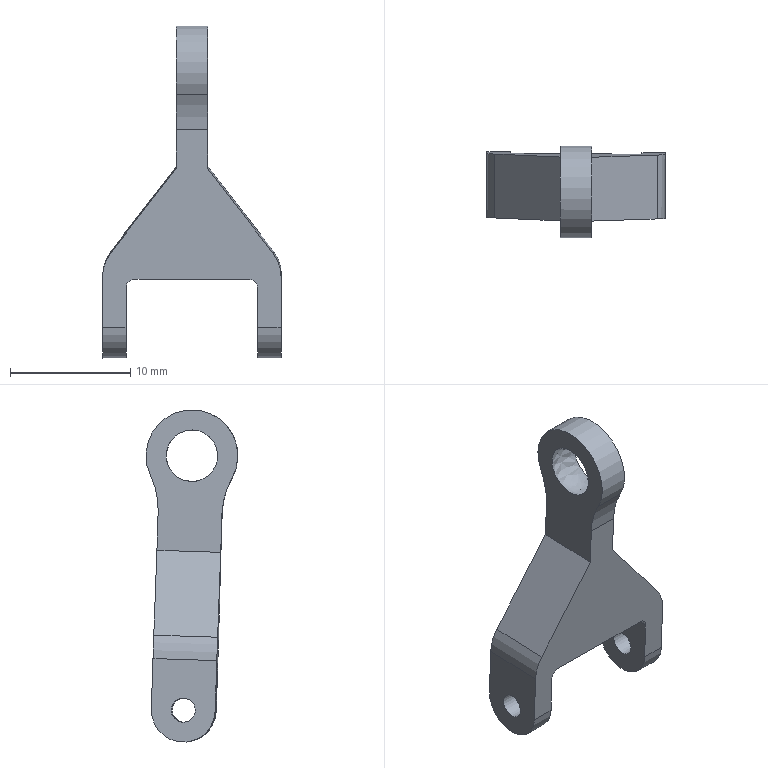Component | NX | ROTATING_ROD | 1 solid | 24 faces | volume 716 mm3 | plane 12 | cylinder 11 | sphere 1 | commonest cylinder face diameters 1.323 x2 6.35 x2 12.7 x2 5.3 x2 2 x2 7.62 x1